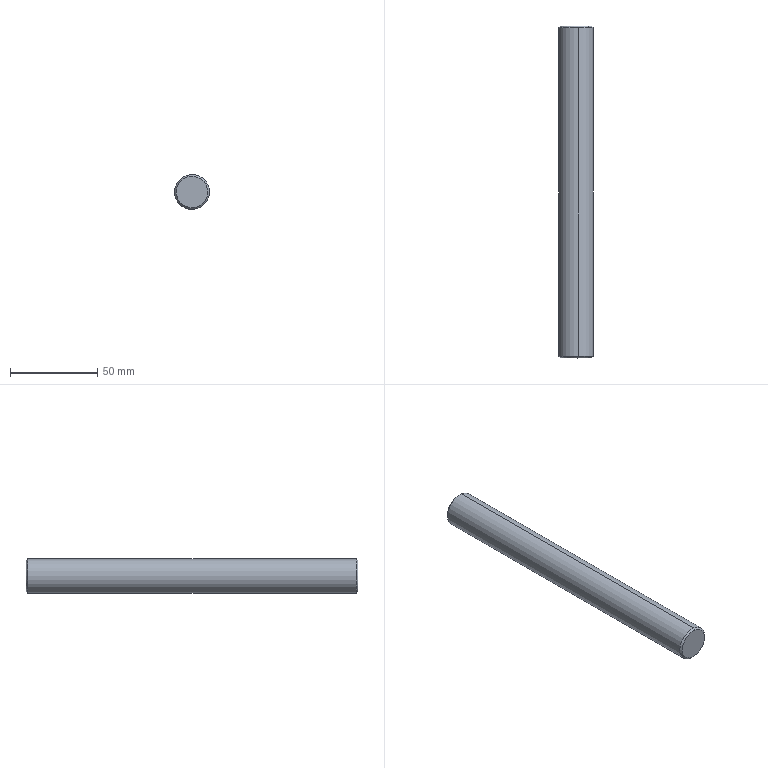Component | SolidWorks | J-007-1 | 1 solid | 12 faces | box 20 x 190 x 20 mm | volume 59325 mm3 | cone 6 | cylinder 4 | plane 2 | commonest cylinder face diameters 5 x2 20 x2 | material 45
build123d program:
from build123d import *

# Parameters (mm, degrees)
SKETCH1_R             = 10
BOSS_EXTRUDE1_DEPTH   = 190
M6_TAPPED_HOLE1_D     = 5
M6_TAPPED_HOLE1_DEPTH = 15
M6_TAPPED_HOLE1_TIP   = 1.502
CHAMFER1_SIZE         = 1
CHAMFER2_SIZE         = 1


with BuildPart() as part:
    # Sketch1 → Boss-Extrude1 (new body)
    with BuildSketch(Plane(origin=(0, 0, 0), x_dir=(1, 0, 0), z_dir=(0, 1, 0))):
        with Locations(Location((0, 0, 0), (0, 0, 270))):
            Circle(SKETCH1_R)
    extrude(amount=BOSS_EXTRUDE1_DEPTH)

    # M6 Tapped Hole1
    with Locations(Plane(origin=(0, 190, 0), x_dir=(1, 0, 0), z_dir=(0, 1, 0))):
        with Locations((0, 0)):
            Hole(M6_TAPPED_HOLE1_D / 2, depth=M6_TAPPED_HOLE1_DEPTH)
            with Locations((0, 0, -(M6_TAPPED_HOLE1_DEPTH + M6_TAPPED_HOLE1_TIP / 2))):  # 118° drill point
                Cone(0, M6_TAPPED_HOLE1_D / 2, M6_TAPPED_HOLE1_TIP, mode=Mode.SUBTRACT)

    # Chamfer1
    chamfer1_edges = [part.edges().sort_by_distance(p)[0] for p in [
        (0, 190, -10),
    ]]
    chamfer(chamfer1_edges, length=CHAMFER1_SIZE)

    # Chamfer2
    chamfer2_edges = [part.edges().sort_by_distance(p)[0] for p in [
        (0, 0, -10),
    ]]
    chamfer(chamfer2_edges, length=CHAMFER2_SIZE)


solid = part.part

# Placed as in the assembly
solid = solid.moved(Location((125.325, 68.019, 297.731), (0, 0, 0)))
STEP:
#1=CARTESIAN_POINT('',(4.883,2.678,11.371));
#2=VERTEX_POINT('',#1);
#3=CARTESIAN_POINT('',(4.985,2.678,12.072));
#4=VERTEX_POINT('',#3);
#5=CARTESIAN_POINT('',(4.934,2.678,11.722));
#6=DIRECTION('',(0.,-1.,0.));
#7=DIRECTION('',(0.1431,0.,0.9897));
#8=AXIS2_PLACEMENT_3D('',#5,#6,#7);
#9=CIRCLE('',#8,0.3543);
#10=EDGE_CURVE('',#2,#4,#9,.T.);
#11=ORIENTED_EDGE('',*,*,#10,.F.);
#12=CARTESIAN_POINT('',(4.878,2.717,11.332));
#13=VERTEX_POINT('',#12);
#14=CARTESIAN_POINT('',(4.878,2.717,11.332));
#15=DIRECTION('',(-0.1012,0.7071,-0.6998));
#16=VECTOR('',#15,39.37);
#17=LINE('',#14,#16);
#18=EDGE_CURVE('',#2,#13,#17,.T.);
#19=ORIENTED_EDGE('',*,*,#18,.T.);
#20=CARTESIAN_POINT('',(4.99,2.717,12.111));
#21=VERTEX_POINT('',#20);
#22=CARTESIAN_POINT('',(4.934,2.717,11.722));
#23=DIRECTION('',(0.,1.,0.));
#24=DIRECTION('',(0.1431,0.,0.9897));
#25=AXIS2_PLACEMENT_3D('',#22,#23,#24);
#26=CIRCLE('',#25,0.3937);
#27=EDGE_CURVE('',#21,#13,#26,.T.);
#28=ORIENTED_EDGE('',*,*,#27,.F.);
#29=CARTESIAN_POINT('',(4.99,2.717,12.111));
#30=DIRECTION('',(0.1012,0.7071,0.6998));
#31=VECTOR('',#30,39.37);
#32=LINE('',#29,#31);
#33=EDGE_CURVE('',#4,#21,#32,.T.);
#34=ORIENTED_EDGE('',*,*,#33,.F.);
#35=EDGE_LOOP('',(#11,#19,#28,#34));
#36=FACE_OUTER_BOUND('',#35,.T.);
#37=CARTESIAN_POINT('',(4.934,2.717,11.722));
#38=DIRECTION('',(0.,1.,0.));
#39=DIRECTION('',(0.1431,0.,0.9897));
#40=AXIS2_PLACEMENT_3D('',#37,#38,#39);
#41=CONICAL_SURFACE('',#40,0.3937,0.7854);
#42=ADVANCED_FACE('',(#36),#41,.T.);
#43=CARTESIAN_POINT('',(4.985,10.158,12.072));
#44=VERTEX_POINT('',#43);
#45=CARTESIAN_POINT('',(4.883,10.158,11.371));
#46=VERTEX_POINT('',#45);
#47=CARTESIAN_POINT('',(4.934,10.158,11.722));
#48=DIRECTION('',(0.,1.,0.));
#49=DIRECTION('',(0.1431,0.,0.9897));
#50=AXIS2_PLACEMENT_3D('',#47,#48,#49);
#51=CIRCLE('',#50,0.3543);
#52=EDGE_CURVE('',#44,#46,#51,.T.);
#53=ORIENTED_EDGE('',*,*,#52,.F.);
#54=CARTESIAN_POINT('',(4.99,10.119,12.111));
#55=VERTEX_POINT('',#54);
#56=CARTESIAN_POINT('',(4.985,10.158,12.072));
#57=DIRECTION('',(0.1012,-0.7071,0.6998));
#58=VECTOR('',#57,39.37);
#59=LINE('',#56,#58);
#60=EDGE_CURVE('',#44,#55,#59,.T.);
#61=ORIENTED_EDGE('',*,*,#60,.T.);
#62=CARTESIAN_POINT('',(4.878,10.119,11.332));
#63=VERTEX_POINT('',#62);
#64=CARTESIAN_POINT('',(4.934,10.119,11.722));
#65=DIRECTION('',(0.,-1.,0.));
#66=DIRECTION('',(0.1431,0.,0.9897));
#67=AXIS2_PLACEMENT_3D('',#64,#65,#66);
#68=CIRCLE('',#67,0.3937);
#69=EDGE_CURVE('',#63,#55,#68,.T.);
#70=ORIENTED_EDGE('',*,*,#69,.F.);
#71=CARTESIAN_POINT('',(4.883,10.158,11.371));
#72=DIRECTION('',(-0.1012,-0.7071,-0.6998));
#73=VECTOR('',#72,39.37);
#74=LINE('',#71,#73);
#75=EDGE_CURVE('',#46,#63,#74,.T.);
#76=ORIENTED_EDGE('',*,*,#75,.F.);
#77=EDGE_LOOP('',(#53,#61,#70,#76));
#78=FACE_OUTER_BOUND('',#77,.T.);
#79=CARTESIAN_POINT('',(4.934,10.158,11.722));
#80=DIRECTION('',(0.,-1.,0.));
#81=DIRECTION('',(-0.1431,0.,-0.9897));
#82=AXIS2_PLACEMENT_3D('',#79,#80,#81);
#83=CONICAL_SURFACE('',#82,0.3543,0.7854);
#84=ADVANCED_FACE('',(#78),#83,.T.);
#85=CARTESIAN_POINT('',(4.92,9.568,11.624));
#86=VERTEX_POINT('',#85);
#87=CARTESIAN_POINT('',(4.948,9.568,11.819));
#88=VERTEX_POINT('',#87);
#89=CARTESIAN_POINT('',(4.934,9.568,11.722));
#90=DIRECTION('',(0.,1.,0.));
#91=DIRECTION('',(0.1431,0.,0.9897));
#92=AXIS2_PLACEMENT_3D('',#89,#90,#91);
#93=CIRCLE('',#92,0.09843);
#94=EDGE_CURVE('',#86,#88,#93,.T.);
#95=ORIENTED_EDGE('',*,*,#94,.F.);
#96=CARTESIAN_POINT('',(4.92,10.158,11.624));
#97=VERTEX_POINT('',#96);
#98=CARTESIAN_POINT('',(4.92,10.158,11.624));
#99=DIRECTION('',(0.,1.,0.));
#100=VECTOR('',#99,39.37);
#101=LINE('',#98,#100);
#102=EDGE_CURVE('',#86,#97,#101,.T.);
#103=ORIENTED_EDGE('',*,*,#102,.T.);
#104=CARTESIAN_POINT('',(4.948,10.158,11.819));
#105=VERTEX_POINT('',#104);
#106=CARTESIAN_POINT('',(4.934,10.158,11.722));
#107=DIRECTION('',(0.,1.,0.));
#108=DIRECTION('',(0.1431,0.,0.9897));
#109=AXIS2_PLACEMENT_3D('',#106,#107,#108);
#110=CIRCLE('',#109,0.09843);
#111=EDGE_CURVE('',#97,#105,#110,.T.);
#112=ORIENTED_EDGE('',*,*,#111,.T.);
#113=CARTESIAN_POINT('',(4.948,10.158,11.819));
#114=DIRECTION('',(0.,1.,0.));
#115=VECTOR('',#114,39.37);
#116=LINE('',#113,#115);
#117=EDGE_CURVE('',#88,#105,#116,.T.);
#118=ORIENTED_EDGE('',*,*,#117,.F.);
#119=EDGE_LOOP('',(#95,#103,#112,#118));
#120=FACE_OUTER_BOUND('',#119,.T.);
#121=CARTESIAN_POINT('',(4.934,10.158,11.722));
#122=DIRECTION('',(0.,1.,0.));
#123=DIRECTION('',(0.1431,0.,0.9897));
#124=AXIS2_PLACEMENT_3D('',#121,#122,#123);
#125=CYLINDRICAL_SURFACE('',#124,0.09843);
#126=ADVANCED_FACE('',(#120),#125,.F.);
#127=CARTESIAN_POINT('',(4.934,9.509,11.722));
#128=VERTEX_POINT('',#127);
#129=CARTESIAN_POINT('',(4.948,9.568,11.819));
#130=DIRECTION('',(0.1226,0.515,0.8484));
#131=VECTOR('',#130,39.37);
#132=LINE('',#129,#131);
#133=EDGE_CURVE('',#128,#88,#132,.T.);
#134=ORIENTED_EDGE('',*,*,#133,.F.);
#135=CARTESIAN_POINT('',(4.92,9.568,11.624));
#136=DIRECTION('',(-0.1226,0.515,-0.8484));
#137=VECTOR('',#136,39.37);
#138=LINE('',#135,#137);
#139=EDGE_CURVE('',#128,#86,#138,.T.);
#140=ORIENTED_EDGE('',*,*,#139,.T.);
#141=ORIENTED_EDGE('',*,*,#94,.T.);
#142=EDGE_LOOP('',(#134,#140,#141));
#143=FACE_OUTER_BOUND('',#142,.T.);
#144=CARTESIAN_POINT('',(4.934,9.568,11.722));
#145=DIRECTION('',(0.,1.,0.));
#146=DIRECTION('',(0.1431,0.,0.9897));
#147=AXIS2_PLACEMENT_3D('',#144,#145,#146);
#148=CONICAL_SURFACE('',#147,0.09843,1.03);
#149=ADVANCED_FACE('',(#143),#148,.F.);
#150=ORIENTED_EDGE('',*,*,#69,.T.);
#151=CARTESIAN_POINT('',(4.99,10.158,12.111));
#152=DIRECTION('',(0.,-1.,0.));
#153=VECTOR('',#152,39.37);
#154=LINE('',#151,#153);
#155=EDGE_CURVE('',#55,#21,#154,.T.);
#156=ORIENTED_EDGE('',*,*,#155,.T.);
#157=ORIENTED_EDGE('',*,*,#27,.T.);
#158=CARTESIAN_POINT('',(4.878,10.158,11.332));
#159=DIRECTION('',(0.,-1.,0.));
#160=VECTOR('',#159,39.37);
#161=LINE('',#158,#160);
#162=EDGE_CURVE('',#63,#13,#161,.T.);
#163=ORIENTED_EDGE('',*,*,#162,.F.);
#164=EDGE_LOOP('',(#150,#156,#157,#163));
#165=FACE_OUTER_BOUND('',#164,.T.);
#166=CARTESIAN_POINT('',(4.934,10.158,11.722));
#167=DIRECTION('',(0.,-1.,0.));
#168=DIRECTION('',(-0.1431,0.,-0.9897));
#169=AXIS2_PLACEMENT_3D('',#166,#167,#168);
#170=CYLINDRICAL_SURFACE('',#169,0.3937);
#171=ADVANCED_FACE('',(#165),#170,.T.);
#172=ORIENTED_EDGE('',*,*,#155,.F.);
#173=CARTESIAN_POINT('',(4.934,10.119,11.722));
#174=DIRECTION('',(0.,-1.,0.));
#175=DIRECTION('',(0.1431,0.,0.9897));
#176=AXIS2_PLACEMENT_3D('',#173,#174,#175);
#177=CIRCLE('',#176,0.3937);
#178=EDGE_CURVE('',#55,#63,#177,.T.);
#179=ORIENTED_EDGE('',*,*,#178,.T.);
#180=ORIENTED_EDGE('',*,*,#162,.T.);
#181=CARTESIAN_POINT('',(4.934,2.717,11.722));
#182=DIRECTION('',(0.,1.,0.));
#183=DIRECTION('',(0.1431,0.,0.9897));
#184=AXIS2_PLACEMENT_3D('',#181,#182,#183);
#185=CIRCLE('',#184,0.3937);
#186=EDGE_CURVE('',#13,#21,#185,.T.);
#187=ORIENTED_EDGE('',*,*,#186,.T.);
#188=EDGE_LOOP('',(#172,#179,#180,#187));
#189=FACE_OUTER_BOUND('',#188,.T.);
#190=CARTESIAN_POINT('',(4.934,10.158,11.722));
#191=DIRECTION('',(0.,-1.,0.));
#192=DIRECTION('',(-0.1431,0.,-0.9897));
#193=AXIS2_PLACEMENT_3D('',#190,#191,#192);
#194=CYLINDRICAL_SURFACE('',#193,0.3937);
#195=ADVANCED_FACE('',(#189),#194,.T.);
#196=CARTESIAN_POINT('',(4.934,10.158,11.722));
#197=DIRECTION('',(0.,1.,0.));
#198=DIRECTION('',(0.1431,0.,0.9897));
#199=AXIS2_PLACEMENT_3D('',#196,#197,#198);
#200=CIRCLE('',#199,0.3543);
#201=EDGE_CURVE('',#46,#44,#200,.T.);
#202=ORIENTED_EDGE('',*,*,#201,.T.);
#203=ORIENTED_EDGE('',*,*,#52,.T.);
#204=EDGE_LOOP('',(#202,#203));
#205=FACE_OUTER_BOUND('',#204,.T.);
#206=CARTESIAN_POINT('',(4.934,10.158,11.722));
#207=DIRECTION('',(0.,1.,0.));
#208=DIRECTION('',(0.1431,0.,0.9897));
#209=AXIS2_PLACEMENT_3D('',#206,#207,#208);
#210=CIRCLE('',#209,0.09843);
#211=EDGE_CURVE('',#105,#97,#210,.T.);
#212=ORIENTED_EDGE('',*,*,#211,.F.);
#213=ORIENTED_EDGE('',*,*,#111,.F.);
#214=EDGE_LOOP('',(#212,#213));
#215=FACE_BOUND('',#214,.T.);
#216=CARTESIAN_POINT('',(4.934,10.158,11.722));
#217=DIRECTION('',(0.,1.,0.));
#218=DIRECTION('',(0.1431,0.,0.9897));
#219=AXIS2_PLACEMENT_3D('',#216,#217,#218);
#220=PLANE('',#219);
#221=ADVANCED_FACE('',(#205,#215),#220,.T.);
#222=CARTESIAN_POINT('',(4.934,2.678,11.722));
#223=DIRECTION('',(0.,-1.,0.));
#224=DIRECTION('',(0.1431,0.,0.9897));
#225=AXIS2_PLACEMENT_3D('',#222,#223,#224);
#226=CIRCLE('',#225,0.3543);
#227=EDGE_CURVE('',#4,#2,#226,.T.);
#228=ORIENTED_EDGE('',*,*,#227,.T.);
#229=ORIENTED_EDGE('',*,*,#10,.T.);
#230=EDGE_LOOP('',(#228,#229));
#231=FACE_OUTER_BOUND('',#230,.T.);
#232=CARTESIAN_POINT('',(4.934,2.678,11.722));
#233=DIRECTION('',(0.,1.,0.));
#234=DIRECTION('',(0.1431,0.,0.9897));
#235=AXIS2_PLACEMENT_3D('',#232,#233,#234);
#236=PLANE('',#235);
#237=ADVANCED_FACE('',(#231),#236,.F.);
#238=ORIENTED_EDGE('',*,*,#139,.F.);
#239=ORIENTED_EDGE('',*,*,#133,.T.);
#240=CARTESIAN_POINT('',(4.934,9.568,11.722));
#241=DIRECTION('',(0.,1.,0.));
#242=DIRECTION('',(0.1431,0.,0.9897));
#243=AXIS2_PLACEMENT_3D('',#240,#241,#242);
#244=CIRCLE('',#243,0.09843);
#245=EDGE_CURVE('',#88,#86,#244,.T.);
#246=ORIENTED_EDGE('',*,*,#245,.T.);
#247=EDGE_LOOP('',(#238,#239,#246));
#248=FACE_OUTER_BOUND('',#247,.T.);
#249=CARTESIAN_POINT('',(4.934,9.568,11.722));
#250=DIRECTION('',(0.,1.,0.));
#251=DIRECTION('',(0.1431,0.,0.9897));
#252=AXIS2_PLACEMENT_3D('',#249,#250,#251);
#253=CONICAL_SURFACE('',#252,0.09843,1.03);
#254=ADVANCED_FACE('',(#248),#253,.F.);
#255=ORIENTED_EDGE('',*,*,#102,.F.);
#256=ORIENTED_EDGE('',*,*,#245,.F.);
#257=ORIENTED_EDGE('',*,*,#117,.T.);
#258=ORIENTED_EDGE('',*,*,#211,.T.);
#259=EDGE_LOOP('',(#255,#256,#257,#258));
#260=FACE_OUTER_BOUND('',#259,.T.);
#261=CARTESIAN_POINT('',(4.934,10.158,11.722));
#262=DIRECTION('',(0.,1.,0.));
#263=DIRECTION('',(0.1431,0.,0.9897));
#264=AXIS2_PLACEMENT_3D('',#261,#262,#263);
#265=CYLINDRICAL_SURFACE('',#264,0.09843);
#266=ADVANCED_FACE('',(#260),#265,.F.);
#267=ORIENTED_EDGE('',*,*,#60,.F.);
#268=ORIENTED_EDGE('',*,*,#201,.F.);
#269=ORIENTED_EDGE('',*,*,#75,.T.);
#270=ORIENTED_EDGE('',*,*,#178,.F.);
#271=EDGE_LOOP('',(#267,#268,#269,#270));
#272=FACE_OUTER_BOUND('',#271,.T.);
#273=CARTESIAN_POINT('',(4.934,10.158,11.722));
#274=DIRECTION('',(0.,-1.,0.));
#275=DIRECTION('',(-0.1431,0.,-0.9897));
#276=AXIS2_PLACEMENT_3D('',#273,#274,#275);
#277=CONICAL_SURFACE('',#276,0.3543,0.7854);
#278=ADVANCED_FACE('',(#272),#277,.T.);
#279=ORIENTED_EDGE('',*,*,#18,.F.);
#280=ORIENTED_EDGE('',*,*,#227,.F.);
#281=ORIENTED_EDGE('',*,*,#33,.T.);
#282=ORIENTED_EDGE('',*,*,#186,.F.);
#283=EDGE_LOOP('',(#279,#280,#281,#282));
#284=FACE_OUTER_BOUND('',#283,.T.);
#285=CARTESIAN_POINT('',(4.934,2.717,11.722));
#286=DIRECTION('',(0.,1.,0.));
#287=DIRECTION('',(0.1431,0.,0.9897));
#288=AXIS2_PLACEMENT_3D('',#285,#286,#287);
#289=CONICAL_SURFACE('',#288,0.3937,0.7854);
#290=ADVANCED_FACE('',(#284),#289,.T.);
#291=CLOSED_SHELL('',(#42,#84,#126,#149,#171,#195,#221,#237,#254,#266,#278,#290));
#292=MANIFOLD_SOLID_BREP('',#291);
#293=CARTESIAN_POINT('',(0.,0.,0.));
#294=DIRECTION('',(0.,0.,1.));
#295=DIRECTION('',(1.,0.,0.));
#296=AXIS2_PLACEMENT_3D('',#293,#294,#295);
#297=(LENGTH_UNIT()NAMED_UNIT(*)SI_UNIT($,.METRE.));
#298=LENGTH_MEASURE_WITH_UNIT(LENGTH_MEASURE(0.0254),#297);
#299=DIMENSIONAL_EXPONENTS(1.,0.,0.,0.,0.,0.,0.);
#300=(CONVERSION_BASED_UNIT('',#298)LENGTH_UNIT()NAMED_UNIT(#299));
#301=UNCERTAINTY_MEASURE_WITH_UNIT(LENGTH_MEASURE(0.00001),#300,'','');
#302=(NAMED_UNIT(*)PLANE_ANGLE_UNIT()SI_UNIT($,.RADIAN.));
#303=(NAMED_UNIT(*)SI_UNIT($,.STERADIAN.)SOLID_ANGLE_UNIT());
#304=(GEOMETRIC_REPRESENTATION_CONTEXT(3)GLOBAL_UNCERTAINTY_ASSIGNED_CONTEXT((#301))GLOBAL_UNIT_ASSIGNED_CONTEXT((#300,#302,#303))REPRESENTATION_CONTEXT('',''));
#305=ADVANCED_BREP_SHAPE_REPRESENTATION('',(#292,#296),#304);
#306=COLOUR_RGB('',0.7922,0.8196,0.9333);
#307=FILL_AREA_STYLE_COLOUR('',#306);
#308=FILL_AREA_STYLE('',(#307));
#309=SURFACE_STYLE_FILL_AREA(#308);
#310=SURFACE_SIDE_STYLE('',(#309));
#311=SURFACE_STYLE_USAGE(.BOTH.,#310);
#312=PRESENTATION_STYLE_ASSIGNMENT((#311));
#313=STYLED_ITEM('',(#312),#292);
#314=(LENGTH_UNIT()NAMED_UNIT(*)SI_UNIT($,.METRE.));
#315=LENGTH_MEASURE_WITH_UNIT(LENGTH_MEASURE(0.0254),#314);
#316=DIMENSIONAL_EXPONENTS(1.,0.,0.,0.,0.,0.,0.);
#317=(CONVERSION_BASED_UNIT('',#315)LENGTH_UNIT()NAMED_UNIT(#316));
#318=UNCERTAINTY_MEASURE_WITH_UNIT(LENGTH_MEASURE(0.00001),#317,'','');
#319=(NAMED_UNIT(*)PLANE_ANGLE_UNIT()SI_UNIT($,.RADIAN.));
#320=(NAMED_UNIT(*)SI_UNIT($,.STERADIAN.)SOLID_ANGLE_UNIT());
#321=(GEOMETRIC_REPRESENTATION_CONTEXT(3)GLOBAL_UNCERTAINTY_ASSIGNED_CONTEXT((#318))GLOBAL_UNIT_ASSIGNED_CONTEXT((#317,#319,#320))REPRESENTATION_CONTEXT('',''));
#322=MECHANICAL_DESIGN_GEOMETRIC_PRESENTATION_REPRESENTATION('',(#313),#321);
#323=PRESENTATION_LAYER_ASSIGNMENT('','',(#313));